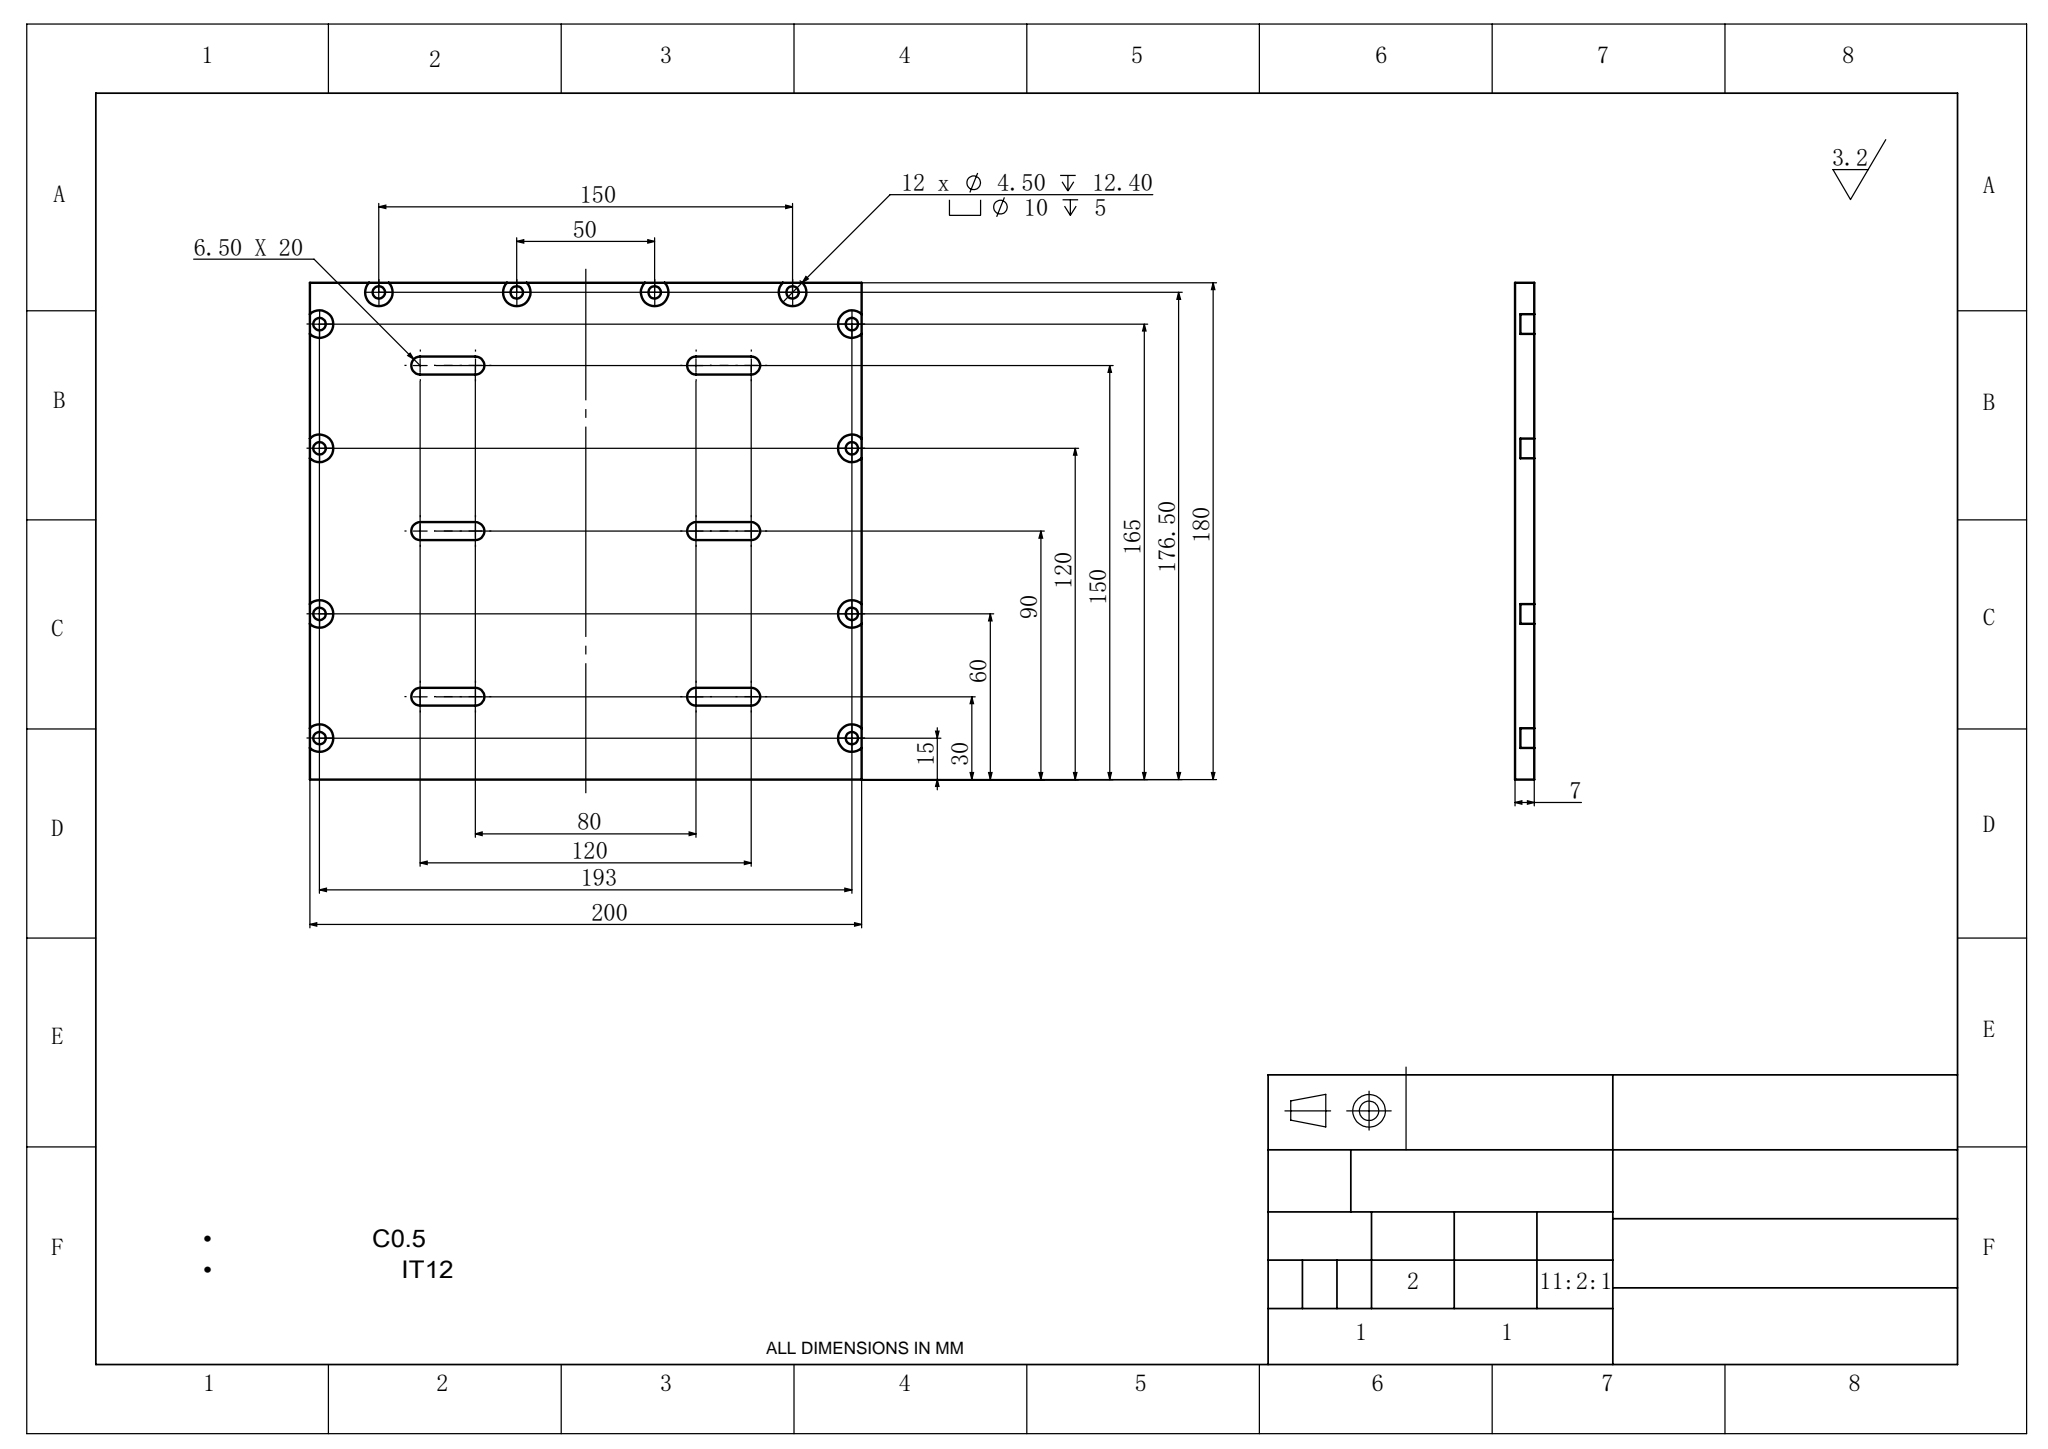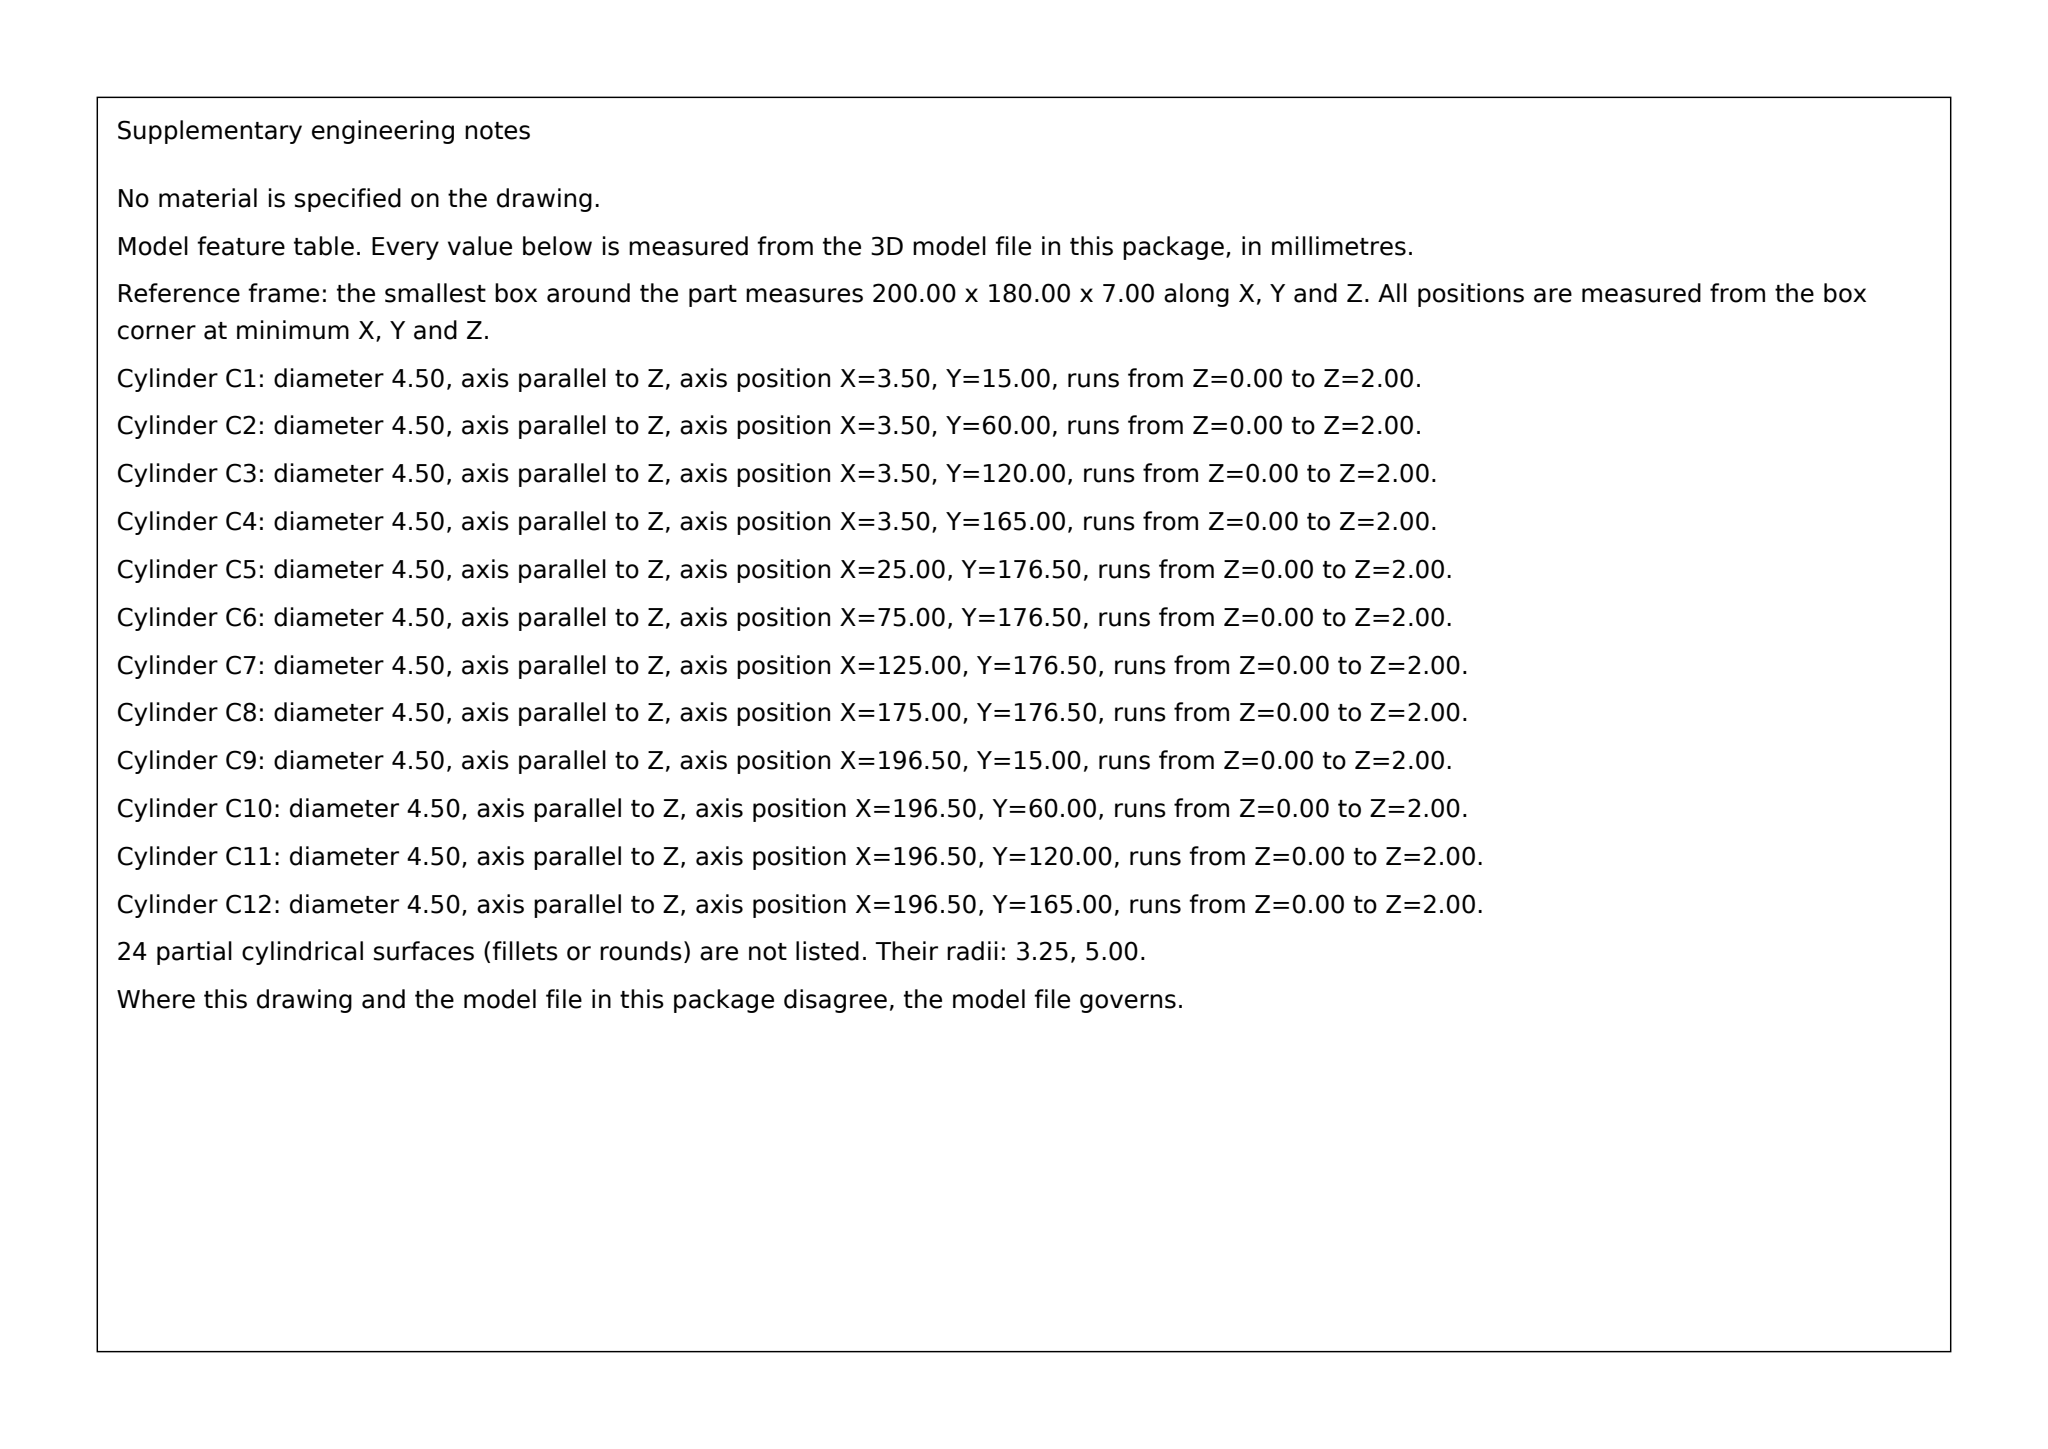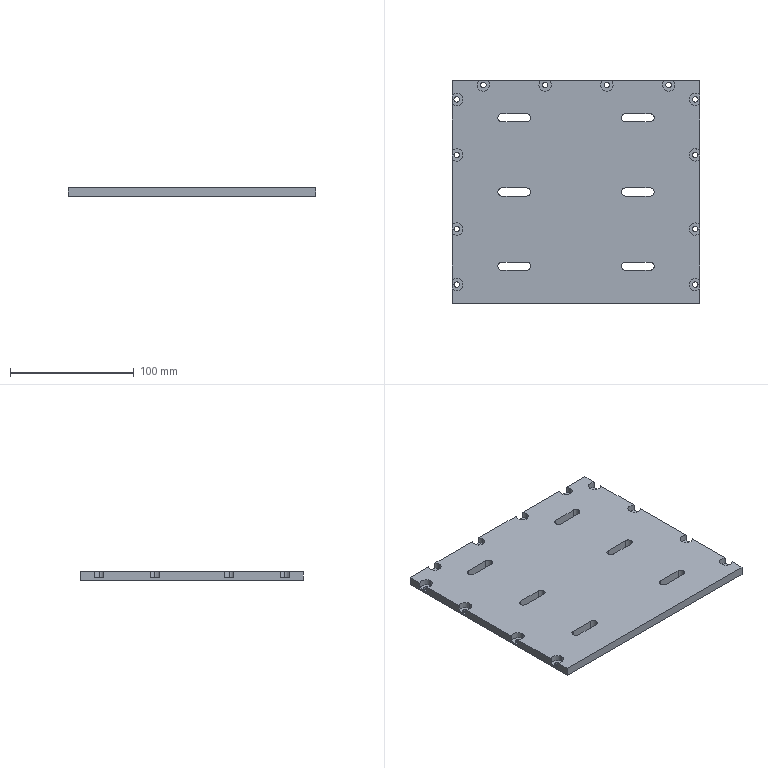Part | SolidWorks | mm | 1 solid | 96 faces | box 200 x 180 x 7 mm | volume 240495 mm3 | cylinder 66 | plane 30 | commonest cylinder face diameters 4.5 x24 10 x24 6.5 x18
build123d program:
from build123d import *

# Parameters (mm, degrees)
SKETCH1_W                                            = 200
SKETCH1_H                                            = 180
BOSS_EXTRUDE1_DEPTH                                  = 7
CUT_EXTRUDE1_DEPTH                                   = 135.718
M4_HEX_HEAD_BOLT_CYLINDRICAL_COUNTERSUNK_D           = 4.5
M4_HEX_HEAD_BOLT_CYLINDRICAL_COUNTERSUNK_DEPTH       = 12.4
M4_HEX_HEAD_BOLT_CYLINDRICAL_COUNTERSUNK_CBORE_D     = 10
M4_HEX_HEAD_BOLT_CYLINDRICAL_COUNTERSUNK_CBORE_DEPTH = 5
M4_HEX_HEAD_BOLT_CYLINDRICAL_COUNTERSUNK_TIP         = 1.352


with BuildPart() as part:
    # Sketch1 → Boss-Extrude1 (new body)
    with BuildSketch(Plane.XY):
        Rectangle(SKETCH1_W, SKETCH1_H)
    extrude(amount=BOSS_EXTRUDE1_DEPTH)

    # Sketch2 → Cut-Extrude1 (cut, through all)
    with BuildSketch(Plane.XY.offset(7)):
        with BuildLine():
            Line((-60, -56.75), (-40, -56.75))
            ThreePointArc((-40, -56.75), (-36.75, -60), (-40, -63.25))
            Line((-40, -63.25), (-60, -63.25))
            ThreePointArc((-60, -63.25), (-63.25, -60), (-60, -56.75))
        make_face()
        with BuildLine():
            Line((-60, 3.25), (-40, 3.25))
            ThreePointArc((-40, 3.25), (-36.75, 0), (-40, -3.25))
            Line((-40, -3.25), (-60, -3.25))
            ThreePointArc((-60, -3.25), (-63.25, 0), (-60, 3.25))
        make_face()
        with BuildLine():
            Line((-60, 63.25), (-40, 63.25))
            ThreePointArc((-40, 63.25), (-36.75, 60), (-40, 56.75))
            Line((-40, 56.75), (-60, 56.75))
            ThreePointArc((-60, 56.75), (-63.25, 60), (-60, 63.25))
        make_face()
        with BuildLine():
            Line((60, 63.25), (40, 63.25))
            ThreePointArc((40, 63.25), (36.75, 60), (40, 56.75))
            Line((40, 56.75), (60, 56.75))
            ThreePointArc((60, 56.75), (63.25, 60), (60, 63.25))
        make_face()
        with BuildLine():
            Line((60, 3.25), (40, 3.25))
            ThreePointArc((40, 3.25), (36.75, 0), (40, -3.25))
            Line((40, -3.25), (60, -3.25))
            ThreePointArc((60, -3.25), (63.25, 0), (60, 3.25))
        make_face()
        with BuildLine():
            Line((60, -56.75), (40, -56.75))
            ThreePointArc((40, -56.75), (36.75, -60), (40, -63.25))
            Line((40, -63.25), (60, -63.25))
            ThreePointArc((60, -63.25), (63.25, -60), (60, -56.75))
        make_face()
    extrude(amount=-CUT_EXTRUDE1_DEPTH, mode=Mode.SUBTRACT)

    # M4 Hex Head Bolt Cylindrical Countersunk
    with Locations(Plane.XY.offset(7)):
        with Locations((-75, 86.5), (-25, 86.5), (25, 86.5), (75, 86.5), (96.5, 75), (96.5, 30), (96.5, -30), (96.5, -75), (-96.5, -75), (-96.5, -30), (-96.5, 30), (-96.5, 75)):
            CounterBoreHole(M4_HEX_HEAD_BOLT_CYLINDRICAL_COUNTERSUNK_D / 2, M4_HEX_HEAD_BOLT_CYLINDRICAL_COUNTERSUNK_CBORE_D / 2, M4_HEX_HEAD_BOLT_CYLINDRICAL_COUNTERSUNK_CBORE_DEPTH, depth=M4_HEX_HEAD_BOLT_CYLINDRICAL_COUNTERSUNK_DEPTH)
            with Locations((0, 0, -(M4_HEX_HEAD_BOLT_CYLINDRICAL_COUNTERSUNK_DEPTH + M4_HEX_HEAD_BOLT_CYLINDRICAL_COUNTERSUNK_TIP / 2))):  # 118° drill point
                Cone(0, M4_HEX_HEAD_BOLT_CYLINDRICAL_COUNTERSUNK_D / 2, M4_HEX_HEAD_BOLT_CYLINDRICAL_COUNTERSUNK_TIP, mode=Mode.SUBTRACT)


solid = part.part